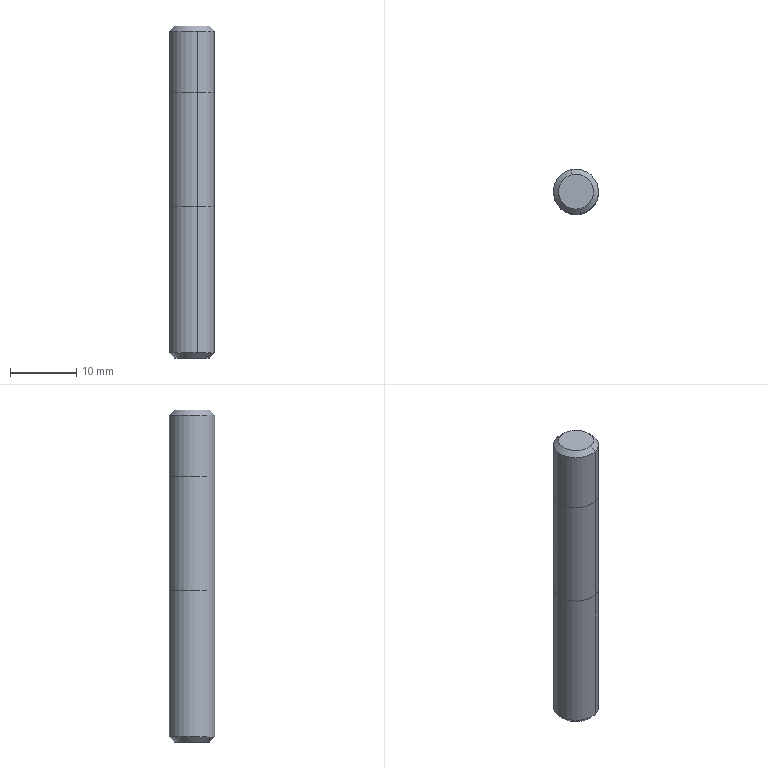Component | SolidWorks | Stud-1 | 3 solids | 16 faces | box 6.8 x 6.8 x 50 mm | volume 1804 mm3 | cylinder 6 | plane 6 | cone 4 | commonest cylinder face diameters 6.8 x6
build123d program:
from build123d import *

# Parameters (mm, degrees)
SKETCH1_4_2_W = 17.23
SKETCH1_4_2_H = 3.4


with BuildPart() as part:
    # Sketch1_4 → Revolve1 (revolve)
    with BuildSketch(Plane.XY, mode=Mode.PRIVATE) as revolve1_sk:
        Polygon((-25, 0), (-15, 0), (-15, 3.4), (-24.23, 3.4), (-25, 2.63), align=None)
        Polygon((2.23, 0), (25, 0), (25, 2.63), (24.23, 3.4), (2.23, 3.4), align=None)
    revolve(revolve1_sk.sketch.rotate(Axis((25, 0, 0), (-1, 0, 0)), 90), axis=Axis((25, 0, 0), (-1, 0, 0)))


with BuildPart() as body_2:
    # Sketch1_4 2 → Revolve2 (revolve)
    with BuildSketch(Plane.XY, mode=Mode.PRIVATE) as revolve2_sk:
        with Locations((-6.385, 1.7)):
            Rectangle(SKETCH1_4_2_W, SKETCH1_4_2_H)
    revolve(revolve2_sk.sketch.rotate(Axis((25, 0, 0), (-1, 0, 0)), 90), axis=Axis((25, 0, 0), (-1, 0, 0)))


solid = Compound([part.part, body_2.part])

# Placed as in the assembly
solid = solid.moved(Location((-105.719, -28.485, 202.01), (0, 90, 0)))
STEP:
#1=COLOUR_RGB('',0.7922,0.8196,0.9333);
#2=FILL_AREA_STYLE_COLOUR('',#1);
#3=FILL_AREA_STYLE('',(#2));
#4=SURFACE_STYLE_FILL_AREA(#3);
#5=SURFACE_SIDE_STYLE('',(#4));
#6=SURFACE_STYLE_USAGE(.BOTH.,#5);
#7=PRESENTATION_STYLE_ASSIGNMENT((#6));
#8=CARTESIAN_POINT('',(-4.132,-1.252,7.865));
#9=VERTEX_POINT('',#8);
#10=CARTESIAN_POINT('',(-4.193,-0.9912,7.865));
#11=VERTEX_POINT('',#10);
#12=CARTESIAN_POINT('',(-4.162,-1.121,7.865));
#13=DIRECTION('',(-0.,0.,-1.));
#14=DIRECTION('',(0.2288,-0.9735,0.));
#15=AXIS2_PLACEMENT_3D('',#12,#13,#14);
#16=CIRCLE('',#15,0.1339);
#17=EDGE_CURVE('',#9,#11,#16,.T.);
#18=ORIENTED_EDGE('',*,*,#17,.T.);
#19=CARTESIAN_POINT('',(-4.193,-0.9912,6.999));
#20=VERTEX_POINT('',#19);
#21=CARTESIAN_POINT('',(-4.193,-0.9912,6.969));
#22=DIRECTION('',(-0.,0.,-1.));
#23=VECTOR('',#22,39.37);
#24=LINE('',#21,#23);
#25=EDGE_CURVE('',#11,#20,#24,.T.);
#26=ORIENTED_EDGE('',*,*,#25,.T.);
#27=CARTESIAN_POINT('',(-4.132,-1.252,6.999));
#28=VERTEX_POINT('',#27);
#29=CARTESIAN_POINT('',(-4.162,-1.121,6.999));
#30=DIRECTION('',(-0.,0.,-1.));
#31=DIRECTION('',(0.2288,-0.9735,0.));
#32=AXIS2_PLACEMENT_3D('',#29,#30,#31);
#33=CIRCLE('',#32,0.1339);
#34=EDGE_CURVE('',#28,#20,#33,.T.);
#35=ORIENTED_EDGE('',*,*,#34,.F.);
#36=CARTESIAN_POINT('',(-4.132,-1.252,6.969));
#37=DIRECTION('',(-0.,0.,-1.));
#38=VECTOR('',#37,39.37);
#39=LINE('',#36,#38);
#40=EDGE_CURVE('',#9,#28,#39,.T.);
#41=ORIENTED_EDGE('',*,*,#40,.F.);
#42=EDGE_LOOP('',(#18,#26,#35,#41));
#43=FACE_OUTER_BOUND('',#42,.T.);
#44=CARTESIAN_POINT('',(-4.162,-1.121,6.969));
#45=DIRECTION('',(-0.,0.,-1.));
#46=DIRECTION('',(0.2288,-0.9735,0.));
#47=AXIS2_PLACEMENT_3D('',#44,#45,#46);
#48=CYLINDRICAL_SURFACE('',#47,0.1339);
#49=ADVANCED_FACE('',(#43),#48,.T.);
#50=CARTESIAN_POINT('',(-4.138,-1.222,6.969));
#51=VERTEX_POINT('',#50);
#52=CARTESIAN_POINT('',(-4.186,-1.021,6.969));
#53=VERTEX_POINT('',#52);
#54=CARTESIAN_POINT('',(-4.162,-1.121,6.969));
#55=DIRECTION('',(-0.,0.,-1.));
#56=DIRECTION('',(0.2288,-0.9735,0.));
#57=AXIS2_PLACEMENT_3D('',#54,#55,#56);
#58=CIRCLE('',#57,0.1035);
#59=EDGE_CURVE('',#51,#53,#58,.T.);
#60=ORIENTED_EDGE('',*,*,#59,.F.);
#61=CARTESIAN_POINT('',(-4.132,-1.252,6.999));
#62=DIRECTION('',(0.1618,-0.6883,0.7071));
#63=VECTOR('',#62,39.37);
#64=LINE('',#61,#63);
#65=EDGE_CURVE('',#51,#28,#64,.T.);
#66=ORIENTED_EDGE('',*,*,#65,.T.);
#67=ORIENTED_EDGE('',*,*,#34,.T.);
#68=CARTESIAN_POINT('',(-4.193,-0.9912,6.999));
#69=DIRECTION('',(-0.1618,0.6883,0.7071));
#70=VECTOR('',#69,39.37);
#71=LINE('',#68,#70);
#72=EDGE_CURVE('',#53,#20,#71,.T.);
#73=ORIENTED_EDGE('',*,*,#72,.F.);
#74=EDGE_LOOP('',(#60,#66,#67,#73));
#75=FACE_OUTER_BOUND('',#74,.T.);
#76=CARTESIAN_POINT('',(-4.162,-1.121,6.999));
#77=DIRECTION('',(0.,-0.,1.));
#78=DIRECTION('',(-0.2288,0.9735,0.));
#79=AXIS2_PLACEMENT_3D('',#76,#77,#78);
#80=CONICAL_SURFACE('',#79,0.1339,0.7854);
#81=ADVANCED_FACE('',(#75),#80,.T.);
#82=CARTESIAN_POINT('',(-4.162,-1.121,6.969));
#83=DIRECTION('',(-0.,0.,-1.));
#84=DIRECTION('',(0.2288,-0.9735,0.));
#85=AXIS2_PLACEMENT_3D('',#82,#83,#84);
#86=CIRCLE('',#85,0.1035);
#87=EDGE_CURVE('',#53,#51,#86,.T.);
#88=ORIENTED_EDGE('',*,*,#87,.T.);
#89=ORIENTED_EDGE('',*,*,#59,.T.);
#90=EDGE_LOOP('',(#88,#89));
#91=FACE_OUTER_BOUND('',#90,.T.);
#92=CARTESIAN_POINT('',(-4.162,-1.121,6.969));
#93=DIRECTION('',(0.,-0.,1.));
#94=DIRECTION('',(-0.2288,0.9735,0.));
#95=AXIS2_PLACEMENT_3D('',#92,#93,#94);
#96=PLANE('',#95);
#97=ADVANCED_FACE('',(#91),#96,.F.);
#98=ORIENTED_EDGE('',*,*,#65,.F.);
#99=ORIENTED_EDGE('',*,*,#87,.F.);
#100=ORIENTED_EDGE('',*,*,#72,.T.);
#101=CARTESIAN_POINT('',(-4.162,-1.121,6.999));
#102=DIRECTION('',(-0.,0.,-1.));
#103=DIRECTION('',(0.2288,-0.9735,0.));
#104=AXIS2_PLACEMENT_3D('',#101,#102,#103);
#105=CIRCLE('',#104,0.1339);
#106=EDGE_CURVE('',#20,#28,#105,.T.);
#107=ORIENTED_EDGE('',*,*,#106,.T.);
#108=EDGE_LOOP('',(#98,#99,#100,#107));
#109=FACE_OUTER_BOUND('',#108,.T.);
#110=CARTESIAN_POINT('',(-4.162,-1.121,6.999));
#111=DIRECTION('',(0.,-0.,1.));
#112=DIRECTION('',(-0.2288,0.9735,0.));
#113=AXIS2_PLACEMENT_3D('',#110,#111,#112);
#114=CONICAL_SURFACE('',#113,0.1339,0.7854);
#115=ADVANCED_FACE('',(#109),#114,.T.);
#116=ORIENTED_EDGE('',*,*,#25,.F.);
#117=CARTESIAN_POINT('',(-4.162,-1.121,7.865));
#118=DIRECTION('',(-0.,0.,-1.));
#119=DIRECTION('',(0.2288,-0.9735,0.));
#120=AXIS2_PLACEMENT_3D('',#117,#118,#119);
#121=CIRCLE('',#120,0.1339);
#122=EDGE_CURVE('',#11,#9,#121,.T.);
#123=ORIENTED_EDGE('',*,*,#122,.T.);
#124=ORIENTED_EDGE('',*,*,#40,.T.);
#125=ORIENTED_EDGE('',*,*,#106,.F.);
#126=EDGE_LOOP('',(#116,#123,#124,#125));
#127=FACE_OUTER_BOUND('',#126,.T.);
#128=CARTESIAN_POINT('',(-4.162,-1.121,6.969));
#129=DIRECTION('',(-0.,0.,-1.));
#130=DIRECTION('',(0.2288,-0.9735,0.));
#131=AXIS2_PLACEMENT_3D('',#128,#129,#130);
#132=CYLINDRICAL_SURFACE('',#131,0.1339);
#133=ADVANCED_FACE('',(#127),#132,.T.);
#134=ORIENTED_EDGE('',*,*,#17,.F.);
#135=ORIENTED_EDGE('',*,*,#122,.F.);
#136=EDGE_LOOP('',(#134,#135));
#137=FACE_OUTER_BOUND('',#136,.T.);
#138=CARTESIAN_POINT('',(-4.162,-1.121,7.865));
#139=DIRECTION('',(0.,-0.,1.));
#140=DIRECTION('',(-0.2288,0.9735,0.));
#141=AXIS2_PLACEMENT_3D('',#138,#139,#140);
#142=PLANE('',#141);
#143=ADVANCED_FACE('',(#137),#142,.T.);
#144=CLOSED_SHELL('',(#49,#81,#97,#115,#133,#143));
#145=MANIFOLD_SOLID_BREP('',#144);
#146=STYLED_ITEM('',(#7),#145);
#147=(LENGTH_UNIT()NAMED_UNIT(*)SI_UNIT($,.METRE.));
#148=LENGTH_MEASURE_WITH_UNIT(LENGTH_MEASURE(0.0254),#147);
#149=DIMENSIONAL_EXPONENTS(1.,0.,0.,0.,0.,0.,0.);
#150=(CONVERSION_BASED_UNIT('',#148)LENGTH_UNIT()NAMED_UNIT(#149));
#151=UNCERTAINTY_MEASURE_WITH_UNIT(LENGTH_MEASURE(0.00001),#150,'','');
#152=(NAMED_UNIT(*)PLANE_ANGLE_UNIT()SI_UNIT($,.RADIAN.));
#153=(NAMED_UNIT(*)SI_UNIT($,.STERADIAN.)SOLID_ANGLE_UNIT());
#154=(GEOMETRIC_REPRESENTATION_CONTEXT(3)GLOBAL_UNCERTAINTY_ASSIGNED_CONTEXT((#151))GLOBAL_UNIT_ASSIGNED_CONTEXT((#150,#152,#153))REPRESENTATION_CONTEXT('',''));
#155=MECHANICAL_DESIGN_GEOMETRIC_PRESENTATION_REPRESENTATION('',(#146),#154);
#156=PRESENTATION_LAYER_ASSIGNMENT('','',(#146));
#157=COLOUR_RGB('',0.7922,0.8196,0.9333);
#158=FILL_AREA_STYLE_COLOUR('',#157);
#159=FILL_AREA_STYLE('',(#158));
#160=SURFACE_STYLE_FILL_AREA(#159);
#161=SURFACE_SIDE_STYLE('',(#160));
#162=SURFACE_STYLE_USAGE(.BOTH.,#161);
#163=PRESENTATION_STYLE_ASSIGNMENT((#162));
#164=CARTESIAN_POINT('',(-4.138,-1.222,8.937));
#165=VERTEX_POINT('',#164);
#166=CARTESIAN_POINT('',(-4.186,-1.021,8.937));
#167=VERTEX_POINT('',#166);
#168=CARTESIAN_POINT('',(-4.162,-1.121,8.937));
#169=DIRECTION('',(-0.,0.,-1.));
#170=DIRECTION('',(0.2288,-0.9735,0.));
#171=AXIS2_PLACEMENT_3D('',#168,#169,#170);
#172=CIRCLE('',#171,0.1035);
#173=EDGE_CURVE('',#165,#167,#172,.T.);
#174=ORIENTED_EDGE('',*,*,#173,.T.);
#175=CARTESIAN_POINT('',(-4.193,-0.9912,8.907));
#176=VERTEX_POINT('',#175);
#177=CARTESIAN_POINT('',(-4.186,-1.021,8.937));
#178=DIRECTION('',(-0.1618,0.6883,-0.7071));
#179=VECTOR('',#178,39.37);
#180=LINE('',#177,#179);
#181=EDGE_CURVE('',#167,#176,#180,.T.);
#182=ORIENTED_EDGE('',*,*,#181,.T.);
#183=CARTESIAN_POINT('',(-4.132,-1.252,8.907));
#184=VERTEX_POINT('',#183);
#185=CARTESIAN_POINT('',(-4.162,-1.121,8.907));
#186=DIRECTION('',(-0.,0.,-1.));
#187=DIRECTION('',(0.2288,-0.9735,0.));
#188=AXIS2_PLACEMENT_3D('',#185,#186,#187);
#189=CIRCLE('',#188,0.1339);
#190=EDGE_CURVE('',#184,#176,#189,.T.);
#191=ORIENTED_EDGE('',*,*,#190,.F.);
#192=CARTESIAN_POINT('',(-4.138,-1.222,8.937));
#193=DIRECTION('',(0.1618,-0.6883,-0.7071));
#194=VECTOR('',#193,39.37);
#195=LINE('',#192,#194);
#196=EDGE_CURVE('',#165,#184,#195,.T.);
#197=ORIENTED_EDGE('',*,*,#196,.F.);
#198=EDGE_LOOP('',(#174,#182,#191,#197));
#199=FACE_OUTER_BOUND('',#198,.T.);
#200=CARTESIAN_POINT('',(-4.162,-1.121,8.937));
#201=DIRECTION('',(-0.,0.,-1.));
#202=DIRECTION('',(0.2288,-0.9735,0.));
#203=AXIS2_PLACEMENT_3D('',#200,#201,#202);
#204=CONICAL_SURFACE('',#203,0.1035,0.7854);
#205=ADVANCED_FACE('',(#199),#204,.T.);
#206=ORIENTED_EDGE('',*,*,#190,.T.);
#207=CARTESIAN_POINT('',(-4.193,-0.9912,8.544));
#208=VERTEX_POINT('',#207);
#209=CARTESIAN_POINT('',(-4.193,-0.9912,6.969));
#210=DIRECTION('',(-0.,0.,-1.));
#211=VECTOR('',#210,39.37);
#212=LINE('',#209,#211);
#213=EDGE_CURVE('',#176,#208,#212,.T.);
#214=ORIENTED_EDGE('',*,*,#213,.T.);
#215=CARTESIAN_POINT('',(-4.132,-1.252,8.544));
#216=VERTEX_POINT('',#215);
#217=CARTESIAN_POINT('',(-4.162,-1.121,8.544));
#218=DIRECTION('',(-0.,0.,-1.));
#219=DIRECTION('',(0.2288,-0.9735,0.));
#220=AXIS2_PLACEMENT_3D('',#217,#218,#219);
#221=CIRCLE('',#220,0.1339);
#222=EDGE_CURVE('',#216,#208,#221,.T.);
#223=ORIENTED_EDGE('',*,*,#222,.F.);
#224=CARTESIAN_POINT('',(-4.132,-1.252,6.969));
#225=DIRECTION('',(-0.,0.,-1.));
#226=VECTOR('',#225,39.37);
#227=LINE('',#224,#226);
#228=EDGE_CURVE('',#184,#216,#227,.T.);
#229=ORIENTED_EDGE('',*,*,#228,.F.);
#230=EDGE_LOOP('',(#206,#214,#223,#229));
#231=FACE_OUTER_BOUND('',#230,.T.);
#232=CARTESIAN_POINT('',(-4.162,-1.121,6.969));
#233=DIRECTION('',(-0.,0.,-1.));
#234=DIRECTION('',(0.2288,-0.9735,0.));
#235=AXIS2_PLACEMENT_3D('',#232,#233,#234);
#236=CYLINDRICAL_SURFACE('',#235,0.1339);
#237=ADVANCED_FACE('',(#231),#236,.T.);
#238=ORIENTED_EDGE('',*,*,#222,.T.);
#239=CARTESIAN_POINT('',(-4.162,-1.121,8.544));
#240=DIRECTION('',(-0.,0.,-1.));
#241=DIRECTION('',(0.2288,-0.9735,0.));
#242=AXIS2_PLACEMENT_3D('',#239,#240,#241);
#243=CIRCLE('',#242,0.1339);
#244=EDGE_CURVE('',#208,#216,#243,.T.);
#245=ORIENTED_EDGE('',*,*,#244,.T.);
#246=EDGE_LOOP('',(#238,#245));
#247=FACE_OUTER_BOUND('',#246,.T.);
#248=CARTESIAN_POINT('',(-4.162,-1.121,8.544));
#249=DIRECTION('',(0.,-0.,1.));
#250=DIRECTION('',(-0.2288,0.9735,0.));
#251=AXIS2_PLACEMENT_3D('',#248,#249,#250);
#252=PLANE('',#251);
#253=ADVANCED_FACE('',(#247),#252,.F.);
#254=ORIENTED_EDGE('',*,*,#213,.F.);
#255=CARTESIAN_POINT('',(-4.162,-1.121,8.907));
#256=DIRECTION('',(-0.,0.,-1.));
#257=DIRECTION('',(0.2288,-0.9735,0.));
#258=AXIS2_PLACEMENT_3D('',#255,#256,#257);
#259=CIRCLE('',#258,0.1339);
#260=EDGE_CURVE('',#176,#184,#259,.T.);
#261=ORIENTED_EDGE('',*,*,#260,.T.);
#262=ORIENTED_EDGE('',*,*,#228,.T.);
#263=ORIENTED_EDGE('',*,*,#244,.F.);
#264=EDGE_LOOP('',(#254,#261,#262,#263));
#265=FACE_OUTER_BOUND('',#264,.T.);
#266=CARTESIAN_POINT('',(-4.162,-1.121,6.969));
#267=DIRECTION('',(-0.,0.,-1.));
#268=DIRECTION('',(0.2288,-0.9735,0.));
#269=AXIS2_PLACEMENT_3D('',#266,#267,#268);
#270=CYLINDRICAL_SURFACE('',#269,0.1339);
#271=ADVANCED_FACE('',(#265),#270,.T.);
#272=ORIENTED_EDGE('',*,*,#181,.F.);
#273=CARTESIAN_POINT('',(-4.162,-1.121,8.937));
#274=DIRECTION('',(-0.,0.,-1.));
#275=DIRECTION('',(0.2288,-0.9735,0.));
#276=AXIS2_PLACEMENT_3D('',#273,#274,#275);
#277=CIRCLE('',#276,0.1035);
#278=EDGE_CURVE('',#167,#165,#277,.T.);
#279=ORIENTED_EDGE('',*,*,#278,.T.);
#280=ORIENTED_EDGE('',*,*,#196,.T.);
#281=ORIENTED_EDGE('',*,*,#260,.F.);
#282=EDGE_LOOP('',(#272,#279,#280,#281));
#283=FACE_OUTER_BOUND('',#282,.T.);
#284=CARTESIAN_POINT('',(-4.162,-1.121,8.937));
#285=DIRECTION('',(-0.,0.,-1.));
#286=DIRECTION('',(0.2288,-0.9735,0.));
#287=AXIS2_PLACEMENT_3D('',#284,#285,#286);
#288=CONICAL_SURFACE('',#287,0.1035,0.7854);
#289=ADVANCED_FACE('',(#283),#288,.T.);
#290=ORIENTED_EDGE('',*,*,#173,.F.);
#291=ORIENTED_EDGE('',*,*,#278,.F.);
#292=EDGE_LOOP('',(#290,#291));
#293=FACE_OUTER_BOUND('',#292,.T.);
#294=CARTESIAN_POINT('',(-4.162,-1.121,8.937));
#295=DIRECTION('',(-0.,0.,-1.));
#296=DIRECTION('',(0.2288,-0.9735,-0.));
#297=AXIS2_PLACEMENT_3D('',#294,#295,#296);
#298=PLANE('',#297);
#299=ADVANCED_FACE('',(#293),#298,.F.);
#300=CLOSED_SHELL('',(#205,#237,#253,#271,#289,#299));
#301=MANIFOLD_SOLID_BREP('',#300);
#302=STYLED_ITEM('',(#163),#301);
#303=PRESENTATION_LAYER_ASSIGNMENT('','',(#302));
#304=(LENGTH_UNIT()NAMED_UNIT(*)SI_UNIT($,.METRE.));
#305=LENGTH_MEASURE_WITH_UNIT(LENGTH_MEASURE(0.0254),#304);
#306=DIMENSIONAL_EXPONENTS(1.,0.,0.,0.,0.,0.,0.);
#307=(CONVERSION_BASED_UNIT('',#305)LENGTH_UNIT()NAMED_UNIT(#306));
#308=UNCERTAINTY_MEASURE_WITH_UNIT(LENGTH_MEASURE(0.00001),#307,'','');
#309=(NAMED_UNIT(*)PLANE_ANGLE_UNIT()SI_UNIT($,.RADIAN.));
#310=(NAMED_UNIT(*)SI_UNIT($,.STERADIAN.)SOLID_ANGLE_UNIT());
#311=(GEOMETRIC_REPRESENTATION_CONTEXT(3)GLOBAL_UNCERTAINTY_ASSIGNED_CONTEXT((#308))GLOBAL_UNIT_ASSIGNED_CONTEXT((#307,#309,#310))REPRESENTATION_CONTEXT('',''));
#312=MECHANICAL_DESIGN_GEOMETRIC_PRESENTATION_REPRESENTATION('',(#302),#311);
#313=COLOUR_RGB('',0.7922,0.8196,0.9333);
#314=FILL_AREA_STYLE_COLOUR('',#313);
#315=FILL_AREA_STYLE('',(#314));
#316=SURFACE_STYLE_FILL_AREA(#315);
#317=SURFACE_SIDE_STYLE('',(#316));
#318=SURFACE_STYLE_USAGE(.BOTH.,#317);
#319=PRESENTATION_STYLE_ASSIGNMENT((#318));
#320=CARTESIAN_POINT('',(-4.132,-1.252,8.544));
#321=VERTEX_POINT('',#320);
#322=CARTESIAN_POINT('',(-4.193,-0.9912,8.544));
#323=VERTEX_POINT('',#322);
#324=CARTESIAN_POINT('',(-4.162,-1.121,8.544));
#325=DIRECTION('',(-0.,0.,-1.));
#326=DIRECTION('',(0.2288,-0.9735,0.));
#327=AXIS2_PLACEMENT_3D('',#324,#325,#326);
#328=CIRCLE('',#327,0.1339);
#329=EDGE_CURVE('',#321,#323,#328,.T.);
#330=ORIENTED_EDGE('',*,*,#329,.T.);
#331=CARTESIAN_POINT('',(-4.193,-0.9912,7.865));
#332=VERTEX_POINT('',#331);
#333=CARTESIAN_POINT('',(-4.193,-0.9912,6.969));
#334=DIRECTION('',(-0.,0.,-1.));
#335=VECTOR('',#334,39.37);
#336=LINE('',#333,#335);
#337=EDGE_CURVE('',#323,#332,#336,.T.);
#338=ORIENTED_EDGE('',*,*,#337,.T.);
#339=CARTESIAN_POINT('',(-4.132,-1.252,7.865));
#340=VERTEX_POINT('',#339);
#341=CARTESIAN_POINT('',(-4.162,-1.121,7.865));
#342=DIRECTION('',(-0.,0.,-1.));
#343=DIRECTION('',(0.2288,-0.9735,0.));
#344=AXIS2_PLACEMENT_3D('',#341,#342,#343);
#345=CIRCLE('',#344,0.1339);
#346=EDGE_CURVE('',#340,#332,#345,.T.);
#347=ORIENTED_EDGE('',*,*,#346,.F.);
#348=CARTESIAN_POINT('',(-4.132,-1.252,6.969));
#349=DIRECTION('',(-0.,0.,-1.));
#350=VECTOR('',#349,39.37);
#351=LINE('',#348,#350);
#352=EDGE_CURVE('',#321,#340,#351,.T.);
#353=ORIENTED_EDGE('',*,*,#352,.F.);
#354=EDGE_LOOP('',(#330,#338,#347,#353));
#355=FACE_OUTER_BOUND('',#354,.T.);
#356=CARTESIAN_POINT('',(-4.162,-1.121,6.969));
#357=DIRECTION('',(-0.,0.,-1.));
#358=DIRECTION('',(0.2288,-0.9735,0.));
#359=AXIS2_PLACEMENT_3D('',#356,#357,#358);
#360=CYLINDRICAL_SURFACE('',#359,0.1339);
#361=ADVANCED_FACE('',(#355),#360,.T.);
#362=ORIENTED_EDGE('',*,*,#346,.T.);
#363=CARTESIAN_POINT('',(-4.162,-1.121,7.865));
#364=DIRECTION('',(-0.,0.,-1.));
#365=DIRECTION('',(0.2288,-0.9735,0.));
#366=AXIS2_PLACEMENT_3D('',#363,#364,#365);
#367=CIRCLE('',#366,0.1339);
#368=EDGE_CURVE('',#332,#340,#367,.T.);
#369=ORIENTED_EDGE('',*,*,#368,.T.);
#370=EDGE_LOOP('',(#362,#369));
#371=FACE_OUTER_BOUND('',#370,.T.);
#372=CARTESIAN_POINT('',(-4.162,-1.121,7.865));
#373=DIRECTION('',(0.,-0.,1.));
#374=DIRECTION('',(-0.2288,0.9735,0.));
#375=AXIS2_PLACEMENT_3D('',#372,#373,#374);
#376=PLANE('',#375);
#377=ADVANCED_FACE('',(#371),#376,.F.);
#378=ORIENTED_EDGE('',*,*,#337,.F.);
#379=CARTESIAN_POINT('',(-4.162,-1.121,8.544));
#380=DIRECTION('',(-0.,0.,-1.));
#381=DIRECTION('',(0.2288,-0.9735,0.));
#382=AXIS2_PLACEMENT_3D('',#379,#380,#381);
#383=CIRCLE('',#382,0.1339);
#384=EDGE_CURVE('',#323,#321,#383,.T.);
#385=ORIENTED_EDGE('',*,*,#384,.T.);
#386=ORIENTED_EDGE('',*,*,#352,.T.);
#387=ORIENTED_EDGE('',*,*,#368,.F.);
#388=EDGE_LOOP('',(#378,#385,#386,#387));
#389=FACE_OUTER_BOUND('',#388,.T.);
#390=CARTESIAN_POINT('',(-4.162,-1.121,6.969));
#391=DIRECTION('',(-0.,0.,-1.));
#392=DIRECTION('',(0.2288,-0.9735,0.));
#393=AXIS2_PLACEMENT_3D('',#390,#391,#392);
#394=CYLINDRICAL_SURFACE('',#393,0.1339);
#395=ADVANCED_FACE('',(#389),#394,.T.);
#396=ORIENTED_EDGE('',*,*,#329,.F.);
#397=ORIENTED_EDGE('',*,*,#384,.F.);
#398=EDGE_LOOP('',(#396,#397));
#399=FACE_OUTER_BOUND('',#398,.T.);
#400=CARTESIAN_POINT('',(-4.162,-1.121,8.544));
#401=DIRECTION('',(0.,-0.,1.));
#402=DIRECTION('',(-0.2288,0.9735,0.));
#403=AXIS2_PLACEMENT_3D('',#400,#401,#402);
#404=PLANE('',#403);
#405=ADVANCED_FACE('',(#399),#404,.T.);
#406=CLOSED_SHELL('',(#361,#377,#395,#405));
#407=MANIFOLD_SOLID_BREP('',#406);
#408=STYLED_ITEM('',(#319),#407);
#409=(LENGTH_UNIT()NAMED_UNIT(*)SI_UNIT($,.METRE.));
#410=LENGTH_MEASURE_WITH_UNIT(LENGTH_MEASURE(0.0254),#409);
#411=DIMENSIONAL_EXPONENTS(1.,0.,0.,0.,0.,0.,0.);
#412=(CONVERSION_BASED_UNIT('',#410)LENGTH_UNIT()NAMED_UNIT(#411));
#413=UNCERTAINTY_MEASURE_WITH_UNIT(LENGTH_MEASURE(0.00001),#412,'','');
#414=(NAMED_UNIT(*)PLANE_ANGLE_UNIT()SI_UNIT($,.RADIAN.));
#415=(NAMED_UNIT(*)SI_UNIT($,.STERADIAN.)SOLID_ANGLE_UNIT());
#416=(GEOMETRIC_REPRESENTATION_CONTEXT(3)GLOBAL_UNCERTAINTY_ASSIGNED_CONTEXT((#413))GLOBAL_UNIT_ASSIGNED_CONTEXT((#412,#414,#415))REPRESENTATION_CONTEXT('',''));
#417=MECHANICAL_DESIGN_GEOMETRIC_PRESENTATION_REPRESENTATION('',(#408),#416);
#418=CARTESIAN_POINT('',(0.,0.,0.));
#419=DIRECTION('',(0.,0.,1.));
#420=DIRECTION('',(1.,0.,0.));
#421=AXIS2_PLACEMENT_3D('',#418,#419,#420);
#422=(LENGTH_UNIT()NAMED_UNIT(*)SI_UNIT($,.METRE.));
#423=LENGTH_MEASURE_WITH_UNIT(LENGTH_MEASURE(0.0254),#422);
#424=DIMENSIONAL_EXPONENTS(1.,0.,0.,0.,0.,0.,0.);
#425=(CONVERSION_BASED_UNIT('',#423)LENGTH_UNIT()NAMED_UNIT(#424));
#426=UNCERTAINTY_MEASURE_WITH_UNIT(LENGTH_MEASURE(0.00001),#425,'','');
#427=(NAMED_UNIT(*)PLANE_ANGLE_UNIT()SI_UNIT($,.RADIAN.));
#428=(NAMED_UNIT(*)SI_UNIT($,.STERADIAN.)SOLID_ANGLE_UNIT());
#429=(GEOMETRIC_REPRESENTATION_CONTEXT(3)GLOBAL_UNCERTAINTY_ASSIGNED_CONTEXT((#426))GLOBAL_UNIT_ASSIGNED_CONTEXT((#425,#427,#428))REPRESENTATION_CONTEXT('',''));
#430=ADVANCED_BREP_SHAPE_REPRESENTATION('',(#407,#145,#301,#421),#429);
#431=PRESENTATION_LAYER_ASSIGNMENT('','',(#408));